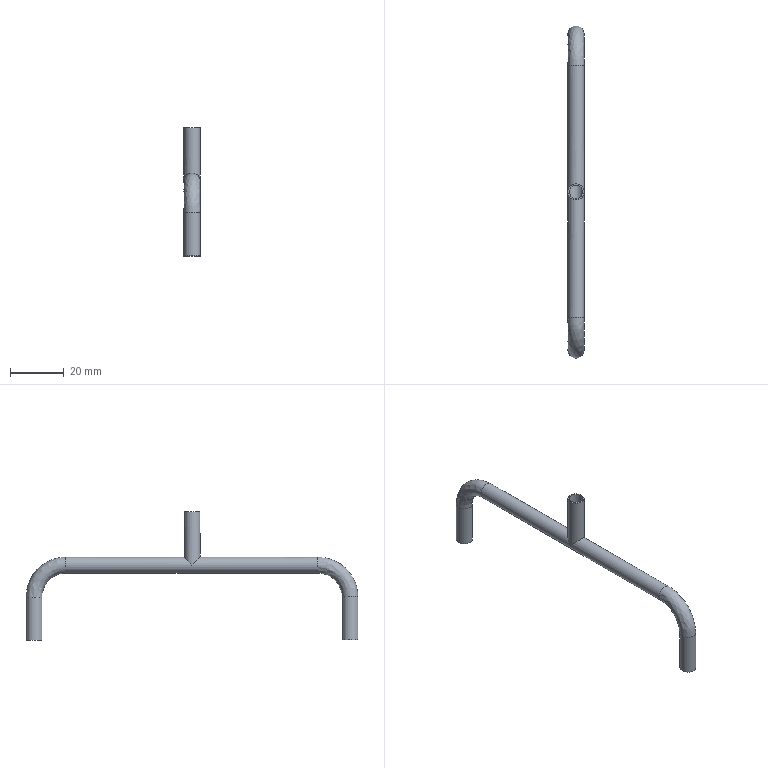Component | NX | PIPE | 1 solid | 15 faces | volume 1557 mm3 | cylinder 8 | other 4 | plane 3 | commonest cylinder face diameters 5 x4 6 x4